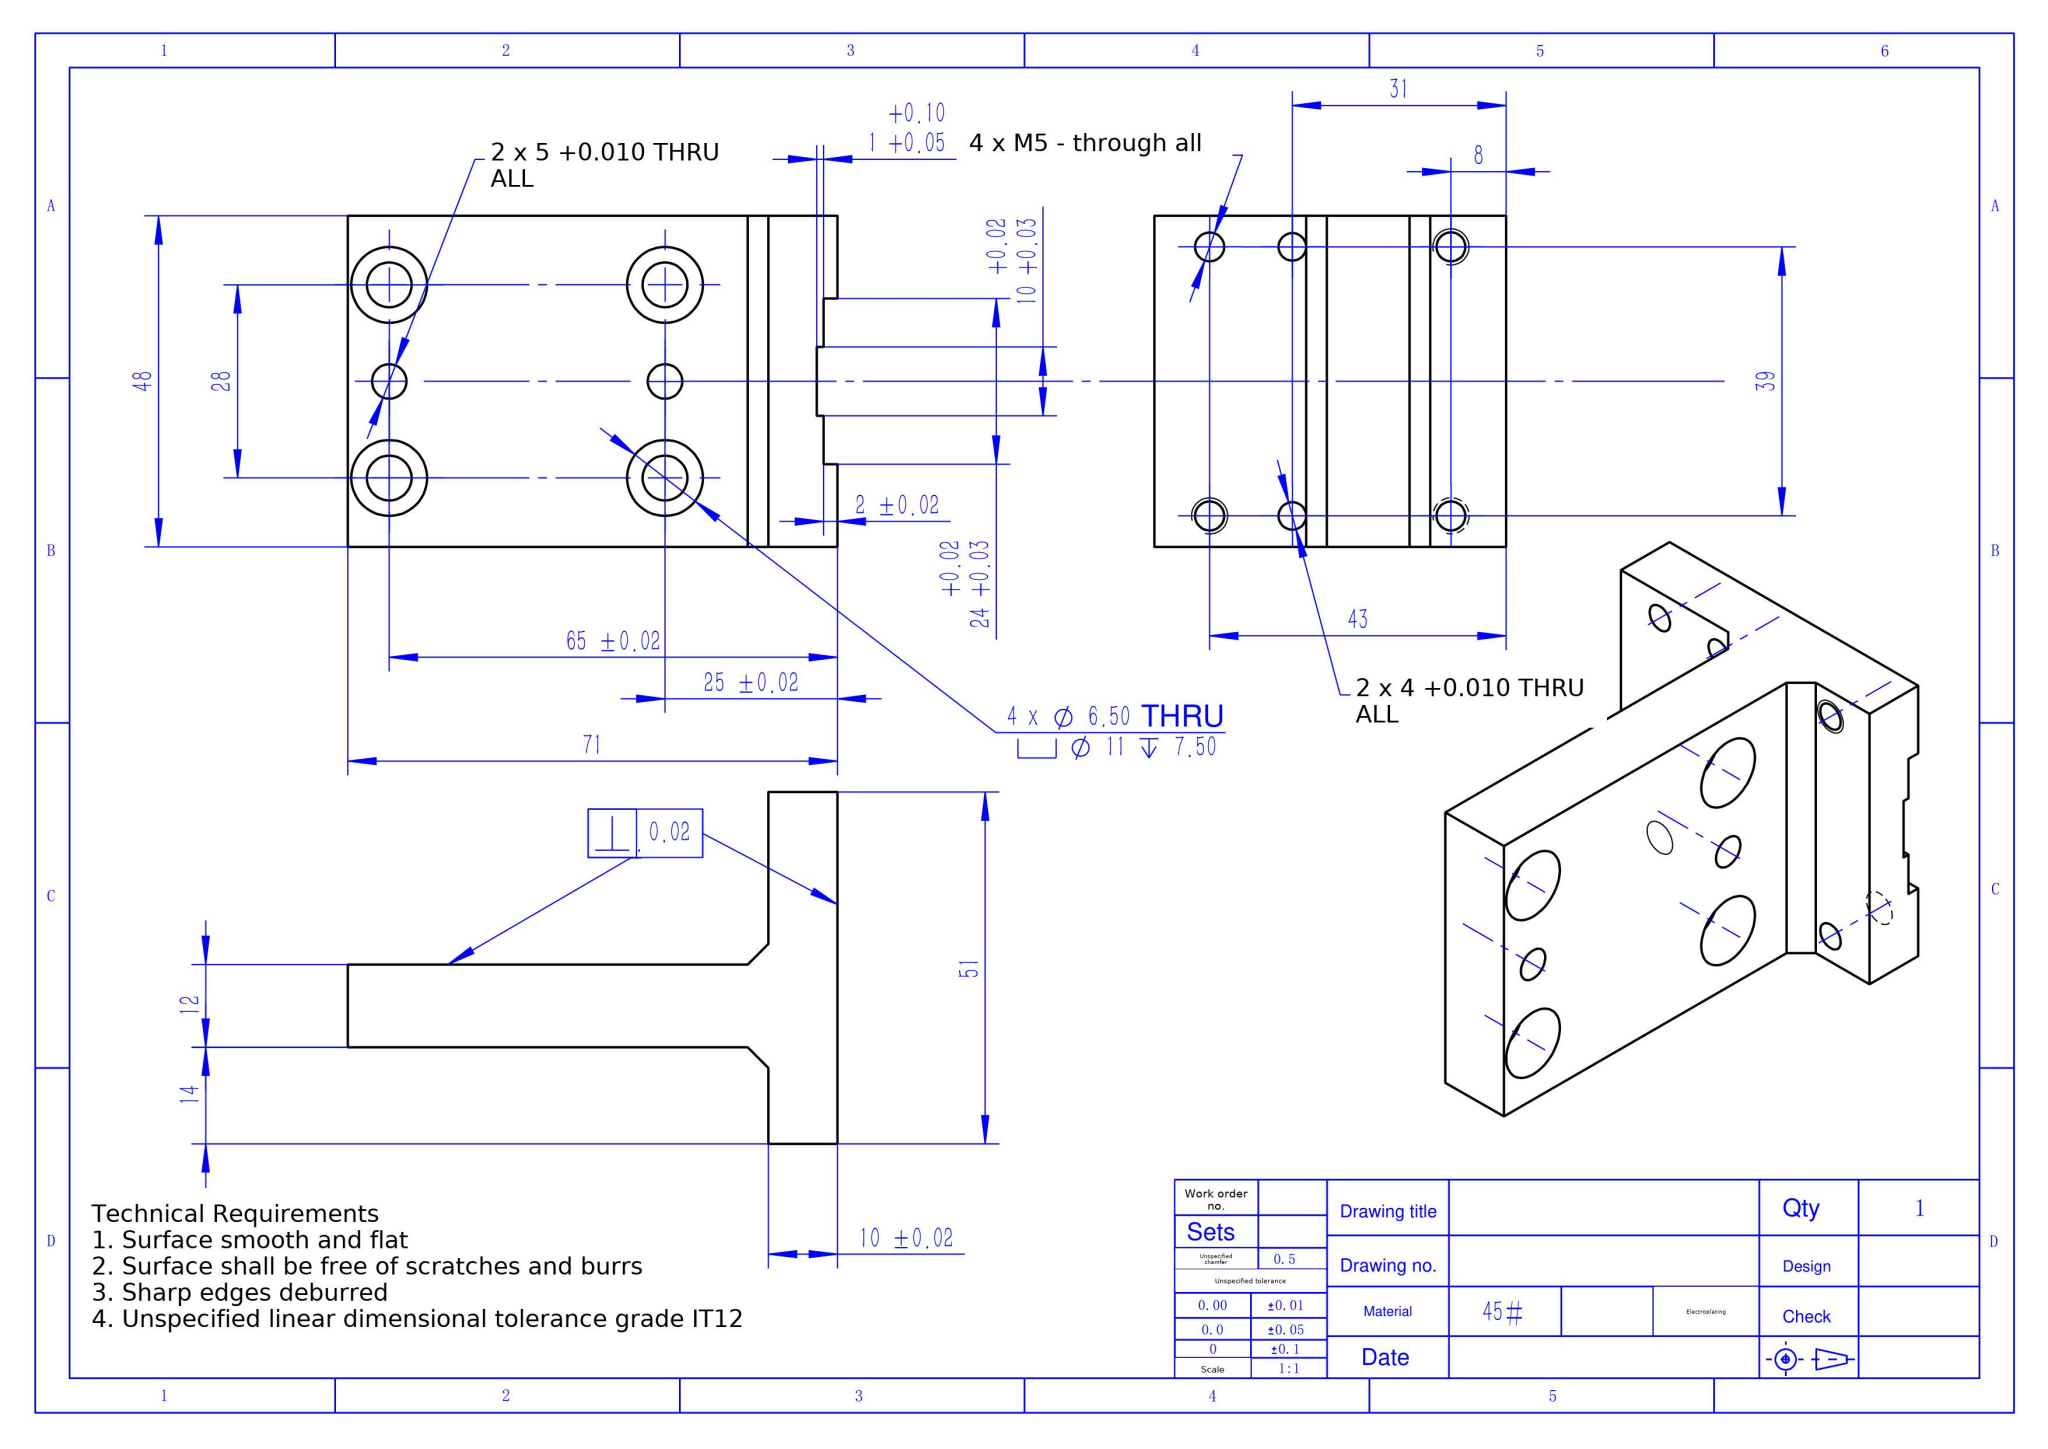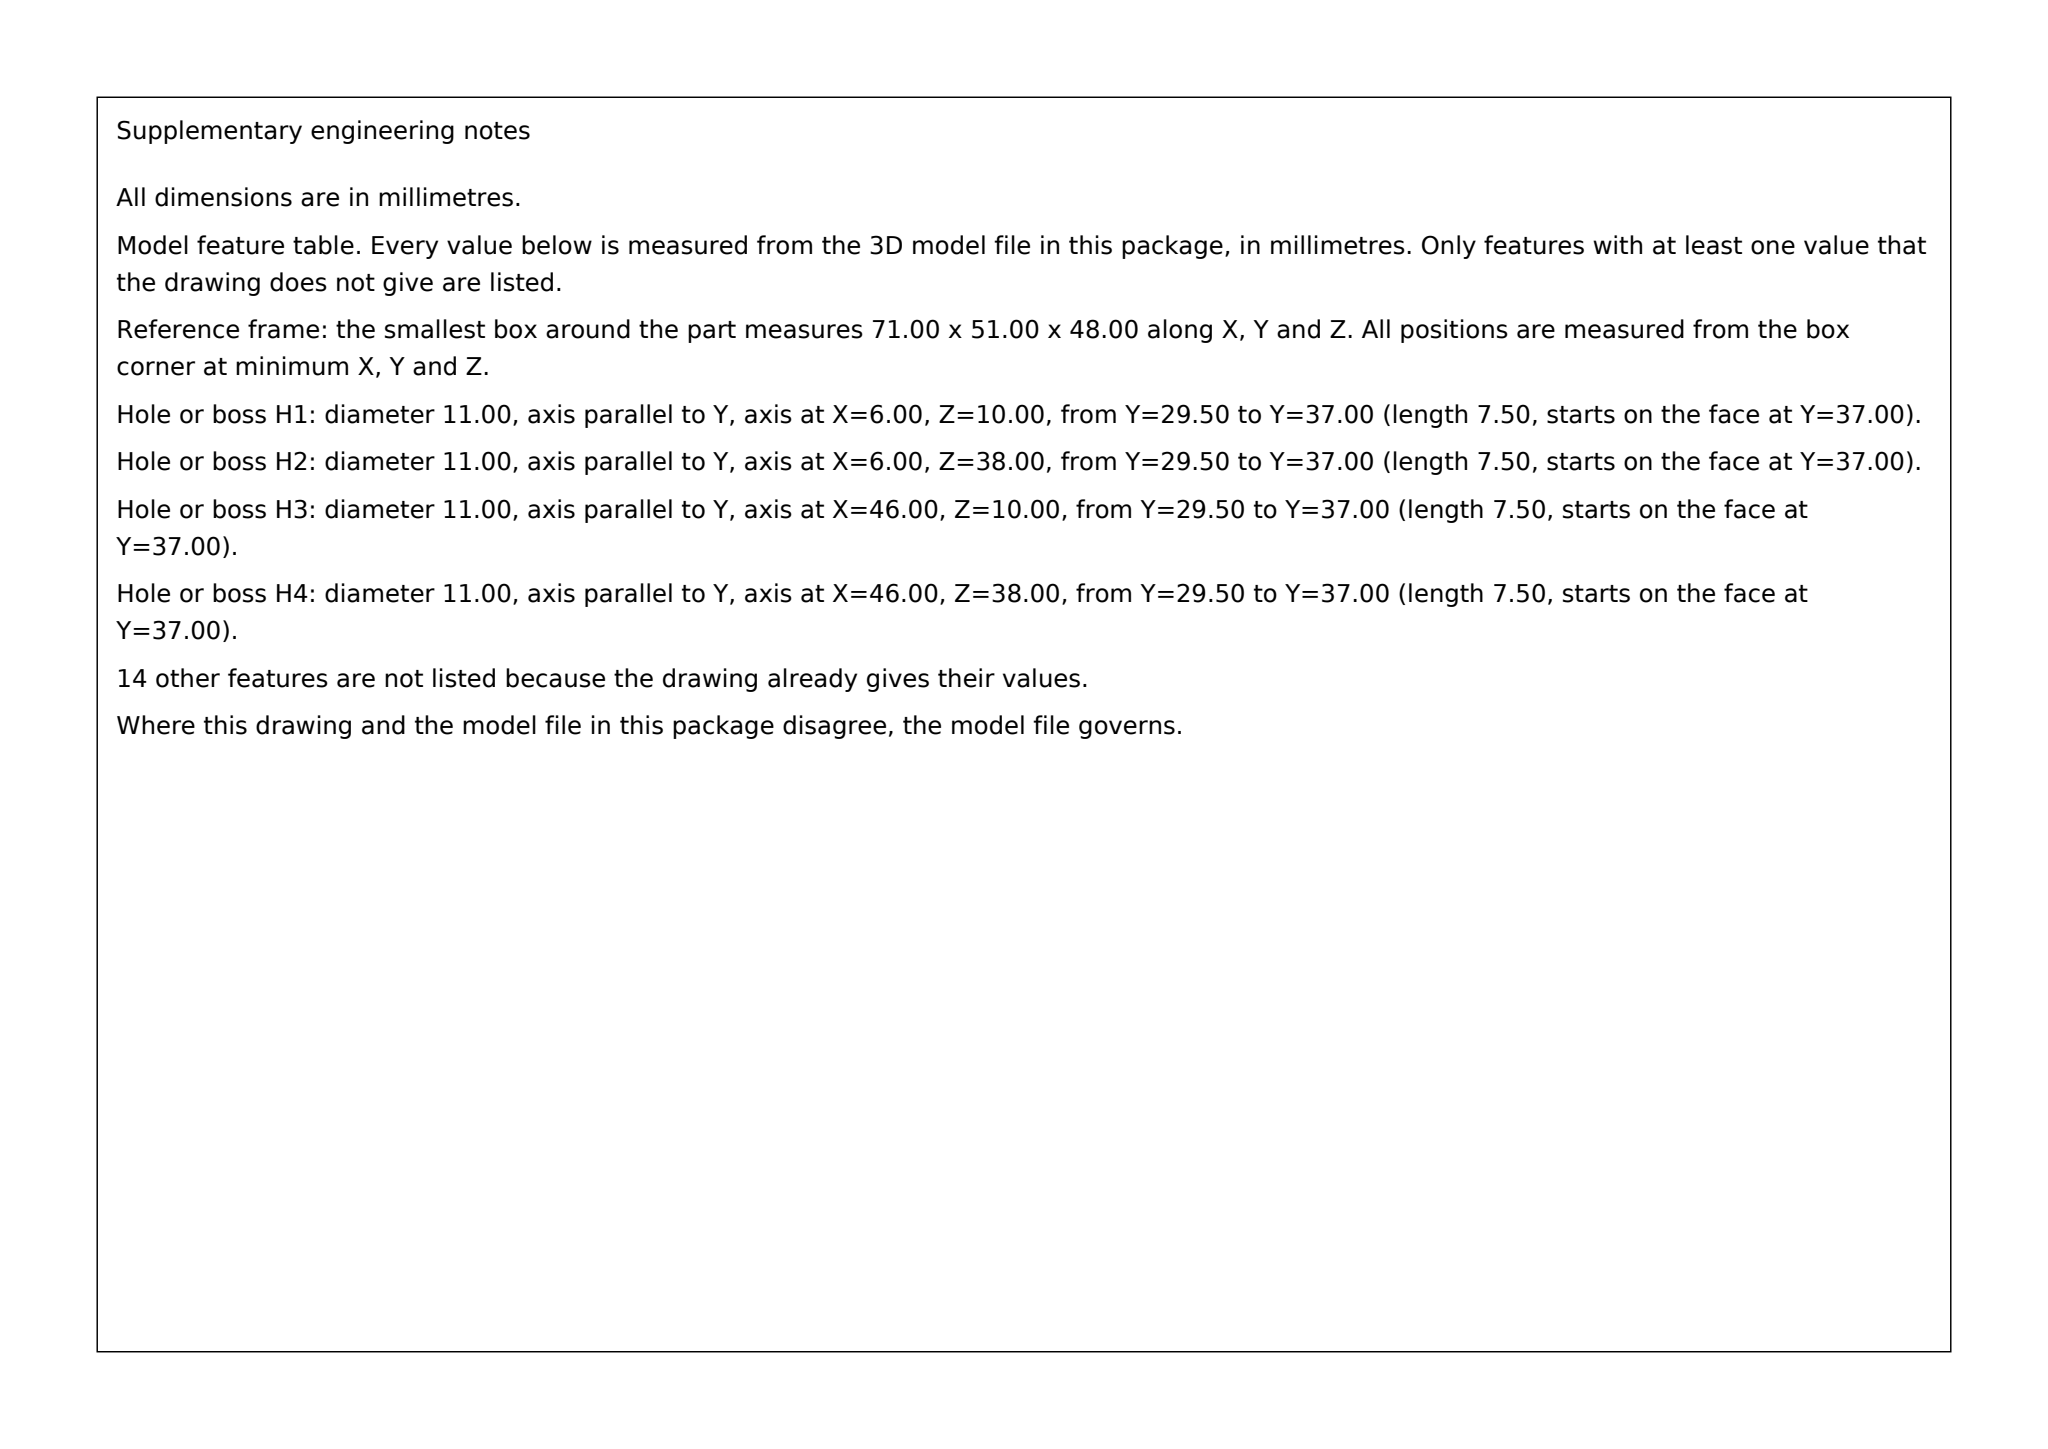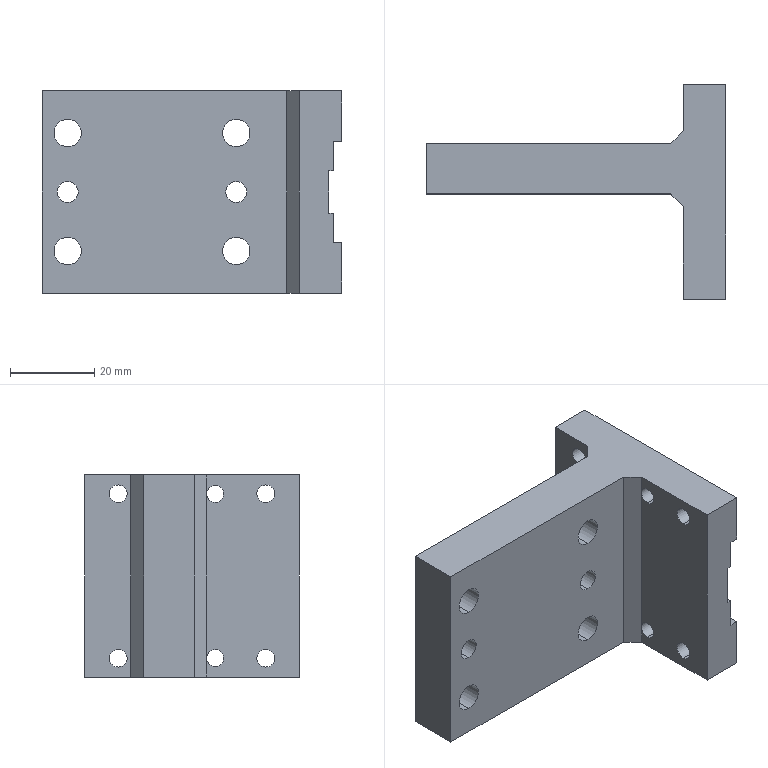Part | SolidWorks | mm | material 45# | 1 solid | 56 faces | box 71 x 51 x 48 mm | volume 52365 mm3 | cylinder 32 | plane 24 | commonest cylinder face diameters 4.2 x8 11 x8 6.5 x8 4 x4 5 x4